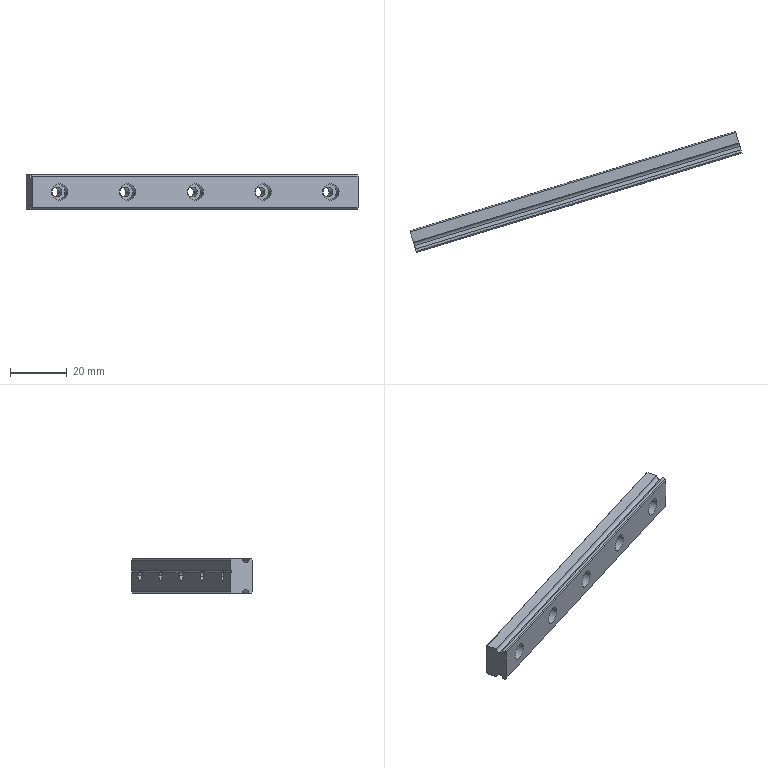Component | SolidWorks | v1ZHXTMGN12HSB1-1_v1ZHXTMGN12H--11SB1-1 | 1 solid | 42 faces | box 117.11 x 42.67 x 12 mm | volume 10165 mm3 | cylinder 24 | plane 18 | commonest cylinder face diameters 6 x10 3.5 x10 2.5 x3 0.6 x1
build123d program:
from build123d import *

# Parameters (mm, degrees)
SKETCH1_W                                           = 12
SKETCH1_H                                           = 120
BOSS_EXTRUDE1_DEPTH                                 = 8
F_2_5_2_5_DIAMETER_HOLE1_D                          = 2.5
F_0_6_0_6_DIAMETER_HOLE1_D                          = 0.6
CYLINDRICAL_COUNTERSUNK_HOLE_FOR_M3_HEX_D           = 3.5
CYLINDRICAL_COUNTERSUNK_HOLE_FOR_M3_HEX_CBORE_D     = 6
CYLINDRICAL_COUNTERSUNK_HOLE_FOR_M3_HEX_CBORE_DEPTH = 3.5
CHAMFER1_SIZE                                       = 0.4


with BuildPart() as part:
    # Sketch1 → Boss-Extrude1 (new body)
    with BuildSketch(Plane.XZ):
        Rectangle(SKETCH1_W, SKETCH1_H)
    extrude(amount=-BOSS_EXTRUDE1_DEPTH)

    # 2.5 _2.5_ Diameter Hole1 (through all)
    with Locations(Plane(origin=(0, 0, -60), x_dir=(-1, 0, 0), z_dir=(0, 0, -1))):
        with Locations((-6, 5.5), (6, 5.5)):
            Hole(F_2_5_2_5_DIAMETER_HOLE1_D / 2)

    # 0.6 _0.6_ Diameter Hole1 (through all)
    with Locations(Plane.XY.offset(60)):
        with Locations((1.5, 0)):
            Hole(F_0_6_0_6_DIAMETER_HOLE1_D / 2)

    # Cylindrical Countersunk Hole for M3 Hex (through all)
    with Locations(Plane(origin=(0, 8, 0), x_dir=(1, 0, 0), z_dir=(0, 1, 0))):
        with Locations((0, -50), (0, -25), (0, 0), (0, 25), (0, 50)):
            CounterBoreHole(CYLINDRICAL_COUNTERSUNK_HOLE_FOR_M3_HEX_D / 2, CYLINDRICAL_COUNTERSUNK_HOLE_FOR_M3_HEX_CBORE_D / 2, CYLINDRICAL_COUNTERSUNK_HOLE_FOR_M3_HEX_CBORE_DEPTH)

    # Chamfer1
    chamfer1_edges = [part.edges().sort_by_distance(p)[0] for p in [
        (-6, 8, 0),
        (6, 8, 0),
        (-6, 0, 0),
        (6, 0, 0),
    ]]
    chamfer(chamfer1_edges, length=CHAMFER1_SIZE)


solid = part.part

# Placed as in the assembly
solid = solid.moved(Location((164.556, -164.917, 407.739), (-90, 73.032, -90)))